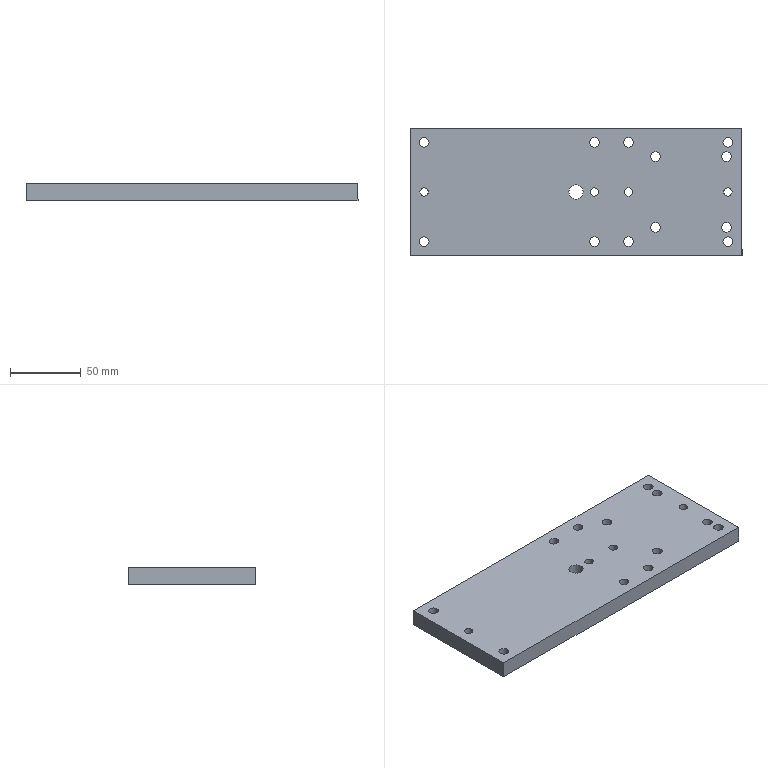Component | SolidWorks | U-AxisSlideMountingPlate-1 | 1 solid | 40 faces | box 234 x 90 x 12 mm | volume 245191 mm3 | cylinder 34 | plane 6 | commonest cylinder face diameters 6.8 x24 6 x8 10 x2 | material Aluminum 6061 (GB)
build123d program:
from build123d import *

# Parameters (mm, degrees)
SKETCH1_W           = 234
SKETCH1_H           = 90
BOSS_EXTRUDE1_DEPTH = 12
SKETCH2_R           = 3
CUT_EXTRUDE1_DEPTH  = 126.929
M8_TAPPED_HOLE1_D   = 6.8
M8_TAPPED_HOLE2_D   = 6.8
SKETCH8_R           = 5
CUT_EXTRUDE2_DEPTH  = 126.929


with BuildPart() as part:
    # Sketch1 → Boss-Extrude1 (new body)
    with BuildSketch(Plane.XY):
        Rectangle(SKETCH1_W, SKETCH1_H)
    extrude(amount=BOSS_EXTRUDE1_DEPTH)

    # Sketch2 → Cut-Extrude1 (cut, through all)
    with BuildSketch(Plane.XY.offset(12)):
        with Locations((-107, 0)):
            Circle(SKETCH2_R)
        with Locations((-37, 0)):
            Circle(SKETCH2_R)
        with Locations((-13, 0)):
            Circle(SKETCH2_R)
        with Locations((107, 0)):
            Circle(SKETCH2_R)
    extrude(amount=-CUT_EXTRUDE1_DEPTH, mode=Mode.SUBTRACT)

    # M8 Tapped Hole1 (through all)
    with Locations(Plane.XY.offset(12)):
        with Locations((-107, 35), (-37, 35), (-37, -35), (-107, -35), (-13, -35), (-13, 35), (107, 35), (107, -35)):
            Hole(M8_TAPPED_HOLE1_D / 2)

    # M8 Tapped Hole2 (through all)
    with Locations(Plane(origin=(0, 0, 0), x_dir=(-1, 0, 0), z_dir=(0, 0, -1))):
        with Locations((56, 25), (56, -25), (106, 25), (106, -25)):
            Hole(M8_TAPPED_HOLE2_D / 2)

    # Sketch8 → Cut-Extrude2 (cut, through all)
    with BuildSketch(Plane.XY.offset(12)):
        Circle(SKETCH8_R)
    extrude(amount=-CUT_EXTRUDE2_DEPTH, mode=Mode.SUBTRACT)


solid = part.part

# Placed as in the assembly
solid = solid.moved(Location((18.729, -71.882, -98.5), (-180, 0, 180)))